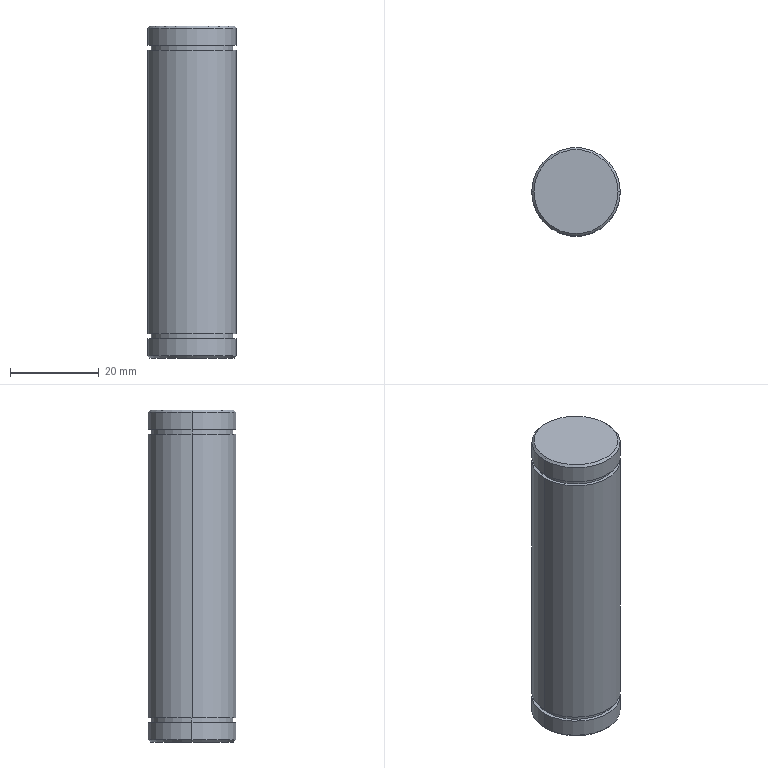Component | SolidWorks | ConnectingPin2-1 | 1 solid | 20 faces | box 20 x 20 x 75 mm | volume 23447 mm3 | cylinder 10 | plane 6 | cone 4 | commonest cylinder face diameters 20 x6 18.5 x4
build123d program:
from build123d import *

# Parameters (mm, degrees)
SKETCH1_R           = 10
BOSS_EXTRUDE1_DEPTH = 37.5
SKETCH2_W           = 1.1
SKETCH2_H           = 0.75
CHAMFER1_SIZE       = 0.5


with BuildPart() as part:
    # Sketch1 → Boss-Extrude1 (new, symmetric)
    with BuildSketch(Plane(origin=(0, 0, 0), x_dir=(0, 0, -1), z_dir=(1, 0, 0))):
        Circle(SKETCH1_R)
    extrude(amount=BOSS_EXTRUDE1_DEPTH, both=True)

    # Sketch2 → Cut-Revolve1 (revolve, cut)
    with BuildSketch(Plane.XY, mode=Mode.PRIVATE) as cut_revolve1_sk:
        with Locations((-32.55, 9.625)):
            Rectangle(SKETCH2_W, SKETCH2_H)
    cut_revolve1 = revolve(cut_revolve1_sk.sketch.rotate(Axis((37.5, 0, 0), (-1, 0, 0)), 90), axis=Axis((37.5, 0, 0), (-1, 0, 0)), mode=Mode.SUBTRACT)

    # Chamfer1
    chamfer1_edges = [part.edges().sort_by_distance(p)[0] for p in [
        (-37.5, 0, 10),
        (37.5, 0, 10),
    ]]
    chamfer(chamfer1_edges, length=CHAMFER1_SIZE)

    # Mirror4: Cut-Revolve1 across plane
    add(cut_revolve1.mirror(Plane(origin=(0, 0, 0), x_dir=(0, 0, 1), z_dir=(1, 0, 0))), mode=Mode.SUBTRACT)


solid = part.part

# Placed as in the assembly
solid = solid.moved(Location((-132.772, 396.234, 900), (0, 90, 0)))
STEP:
#1=COLOUR_RGB('',0.7922,0.8196,0.9333);
#2=FILL_AREA_STYLE_COLOUR('',#1);
#3=FILL_AREA_STYLE('',(#2));
#4=SURFACE_STYLE_FILL_AREA(#3);
#5=SURFACE_SIDE_STYLE('',(#4));
#6=SURFACE_STYLE_USAGE(.BOTH.,#5);
#7=PRESENTATION_STYLE_ASSIGNMENT((#6));
#8=CARTESIAN_POINT('',(-5.621,15.6,36.89));
#9=VERTEX_POINT('',#8);
#10=CARTESIAN_POINT('',(-4.834,15.6,36.89));
#11=VERTEX_POINT('',#10);
#12=CARTESIAN_POINT('',(-5.227,15.6,36.89));
#13=DIRECTION('',(-0.,0.,-1.));
#14=DIRECTION('',(1.,-0.,0.));
#15=AXIS2_PLACEMENT_3D('',#12,#13,#14);
#16=CIRCLE('',#15,0.3937);
#17=EDGE_CURVE('',#9,#11,#16,.T.);
#18=ORIENTED_EDGE('',*,*,#17,.T.);
#19=CARTESIAN_POINT('',(-4.834,15.6,36.736));
#20=VERTEX_POINT('',#19);
#21=CARTESIAN_POINT('',(-4.834,15.6,36.909));
#22=DIRECTION('',(-0.,0.,-1.));
#23=VECTOR('',#22,39.37);
#24=LINE('',#21,#23);
#25=EDGE_CURVE('',#11,#20,#24,.T.);
#26=ORIENTED_EDGE('',*,*,#25,.T.);
#27=CARTESIAN_POINT('',(-5.621,15.6,36.736));
#28=VERTEX_POINT('',#27);
#29=CARTESIAN_POINT('',(-5.227,15.6,36.736));
#30=DIRECTION('',(0.,-0.,1.));
#31=DIRECTION('',(1.,0.,0.));
#32=AXIS2_PLACEMENT_3D('',#29,#30,#31);
#33=CIRCLE('',#32,0.3937);
#34=EDGE_CURVE('',#20,#28,#33,.T.);
#35=ORIENTED_EDGE('',*,*,#34,.T.);
#36=CARTESIAN_POINT('',(-5.621,15.6,36.909));
#37=DIRECTION('',(-0.,0.,-1.));
#38=VECTOR('',#37,39.37);
#39=LINE('',#36,#38);
#40=EDGE_CURVE('',#9,#28,#39,.T.);
#41=ORIENTED_EDGE('',*,*,#40,.F.);
#42=EDGE_LOOP('',(#18,#26,#35,#41));
#43=FACE_OUTER_BOUND('',#42,.T.);
#44=CARTESIAN_POINT('',(-5.227,15.6,36.909));
#45=DIRECTION('',(-0.,0.,-1.));
#46=DIRECTION('',(-1.,0.,0.));
#47=AXIS2_PLACEMENT_3D('',#44,#45,#46);
#48=CYLINDRICAL_SURFACE('',#47,0.3937);
#49=ADVANCED_FACE('',(#43),#48,.T.);
#50=CARTESIAN_POINT('',(-4.853,15.6,36.909));
#51=VERTEX_POINT('',#50);
#52=CARTESIAN_POINT('',(-5.601,15.6,36.909));
#53=VERTEX_POINT('',#52);
#54=CARTESIAN_POINT('',(-5.227,15.6,36.909));
#55=DIRECTION('',(0.,-0.,1.));
#56=DIRECTION('',(1.,0.,0.));
#57=AXIS2_PLACEMENT_3D('',#54,#55,#56);
#58=CIRCLE('',#57,0.374);
#59=EDGE_CURVE('',#51,#53,#58,.T.);
#60=ORIENTED_EDGE('',*,*,#59,.F.);
#61=CARTESIAN_POINT('',(-4.853,15.6,36.909));
#62=DIRECTION('',(0.7071,0.,-0.7071));
#63=VECTOR('',#62,39.37);
#64=LINE('',#61,#63);
#65=EDGE_CURVE('',#51,#11,#64,.T.);
#66=ORIENTED_EDGE('',*,*,#65,.T.);
#67=ORIENTED_EDGE('',*,*,#17,.F.);
#68=CARTESIAN_POINT('',(-5.601,15.6,36.909));
#69=DIRECTION('',(-0.7071,0.,-0.7071));
#70=VECTOR('',#69,39.37);
#71=LINE('',#68,#70);
#72=EDGE_CURVE('',#53,#9,#71,.T.);
#73=ORIENTED_EDGE('',*,*,#72,.F.);
#74=EDGE_LOOP('',(#60,#66,#67,#73));
#75=FACE_OUTER_BOUND('',#74,.T.);
#76=CARTESIAN_POINT('',(-5.227,15.6,36.909));
#77=DIRECTION('',(-0.,0.,-1.));
#78=DIRECTION('',(-1.,0.,0.));
#79=AXIS2_PLACEMENT_3D('',#76,#77,#78);
#80=CONICAL_SURFACE('',#79,0.374,0.7854);
#81=ADVANCED_FACE('',(#75),#80,.T.);
#82=CARTESIAN_POINT('',(-5.591,15.6,36.736));
#83=VERTEX_POINT('',#82);
#84=CARTESIAN_POINT('',(-4.863,15.6,36.736));
#85=VERTEX_POINT('',#84);
#86=CARTESIAN_POINT('',(-5.227,15.6,36.736));
#87=DIRECTION('',(0.,-0.,1.));
#88=DIRECTION('',(1.,0.,0.));
#89=AXIS2_PLACEMENT_3D('',#86,#87,#88);
#90=CIRCLE('',#89,0.3642);
#91=EDGE_CURVE('',#83,#85,#90,.T.);
#92=ORIENTED_EDGE('',*,*,#91,.F.);
#93=CARTESIAN_POINT('',(-5.591,15.6,36.693));
#94=VERTEX_POINT('',#93);
#95=CARTESIAN_POINT('',(-5.591,15.6,36.736));
#96=DIRECTION('',(-0.,0.,-1.));
#97=VECTOR('',#96,39.37);
#98=LINE('',#95,#97);
#99=EDGE_CURVE('',#83,#94,#98,.T.);
#100=ORIENTED_EDGE('',*,*,#99,.T.);
#101=CARTESIAN_POINT('',(-4.863,15.6,36.693));
#102=VERTEX_POINT('',#101);
#103=CARTESIAN_POINT('',(-5.227,15.6,36.693));
#104=DIRECTION('',(0.,-0.,1.));
#105=DIRECTION('',(1.,0.,0.));
#106=AXIS2_PLACEMENT_3D('',#103,#104,#105);
#107=CIRCLE('',#106,0.3642);
#108=EDGE_CURVE('',#94,#102,#107,.T.);
#109=ORIENTED_EDGE('',*,*,#108,.T.);
#110=CARTESIAN_POINT('',(-4.863,15.6,36.736));
#111=DIRECTION('',(-0.,0.,-1.));
#112=VECTOR('',#111,39.37);
#113=LINE('',#110,#112);
#114=EDGE_CURVE('',#85,#102,#113,.T.);
#115=ORIENTED_EDGE('',*,*,#114,.F.);
#116=EDGE_LOOP('',(#92,#100,#109,#115));
#117=FACE_OUTER_BOUND('',#116,.T.);
#118=CARTESIAN_POINT('',(-5.227,15.6,36.736));
#119=DIRECTION('',(-0.,0.,-1.));
#120=DIRECTION('',(1.,0.,0.));
#121=AXIS2_PLACEMENT_3D('',#118,#119,#120);
#122=CYLINDRICAL_SURFACE('',#121,0.3642);
#123=ADVANCED_FACE('',(#117),#122,.T.);
#124=CARTESIAN_POINT('',(-5.601,15.6,33.957));
#125=VERTEX_POINT('',#124);
#126=CARTESIAN_POINT('',(-4.853,15.6,33.957));
#127=VERTEX_POINT('',#126);
#128=CARTESIAN_POINT('',(-5.227,15.6,33.957));
#129=DIRECTION('',(-0.,0.,-1.));
#130=DIRECTION('',(1.,-0.,0.));
#131=AXIS2_PLACEMENT_3D('',#128,#129,#130);
#132=CIRCLE('',#131,0.374);
#133=EDGE_CURVE('',#125,#127,#132,.T.);
#134=ORIENTED_EDGE('',*,*,#133,.F.);
#135=CARTESIAN_POINT('',(-5.621,15.6,33.976));
#136=VERTEX_POINT('',#135);
#137=CARTESIAN_POINT('',(-5.621,15.6,33.976));
#138=DIRECTION('',(-0.7071,0.,0.7071));
#139=VECTOR('',#138,39.37);
#140=LINE('',#137,#139);
#141=EDGE_CURVE('',#125,#136,#140,.T.);
#142=ORIENTED_EDGE('',*,*,#141,.T.);
#143=CARTESIAN_POINT('',(-4.834,15.6,33.976));
#144=VERTEX_POINT('',#143);
#145=CARTESIAN_POINT('',(-5.227,15.6,33.976));
#146=DIRECTION('',(0.,-0.,1.));
#147=DIRECTION('',(1.,0.,0.));
#148=AXIS2_PLACEMENT_3D('',#145,#146,#147);
#149=CIRCLE('',#148,0.3937);
#150=EDGE_CURVE('',#144,#136,#149,.T.);
#151=ORIENTED_EDGE('',*,*,#150,.F.);
#152=CARTESIAN_POINT('',(-4.834,15.6,33.976));
#153=DIRECTION('',(0.7071,-0.,0.7071));
#154=VECTOR('',#153,39.37);
#155=LINE('',#152,#154);
#156=EDGE_CURVE('',#127,#144,#155,.T.);
#157=ORIENTED_EDGE('',*,*,#156,.F.);
#158=EDGE_LOOP('',(#134,#142,#151,#157));
#159=FACE_OUTER_BOUND('',#158,.T.);
#160=CARTESIAN_POINT('',(-5.227,15.6,33.976));
#161=DIRECTION('',(0.,-0.,1.));
#162=DIRECTION('',(1.,0.,0.));
#163=AXIS2_PLACEMENT_3D('',#160,#161,#162);
#164=CONICAL_SURFACE('',#163,0.3937,0.7854);
#165=ADVANCED_FACE('',(#159),#164,.T.);
#166=CARTESIAN_POINT('',(-4.834,15.6,36.693));
#167=VERTEX_POINT('',#166);
#168=CARTESIAN_POINT('',(-5.621,15.6,36.693));
#169=VERTEX_POINT('',#168);
#170=CARTESIAN_POINT('',(-5.227,15.6,36.693));
#171=DIRECTION('',(0.,-0.,1.));
#172=DIRECTION('',(1.,0.,0.));
#173=AXIS2_PLACEMENT_3D('',#170,#171,#172);
#174=CIRCLE('',#173,0.3937);
#175=EDGE_CURVE('',#167,#169,#174,.T.);
#176=ORIENTED_EDGE('',*,*,#175,.F.);
#177=CARTESIAN_POINT('',(-4.834,15.6,34.173));
#178=VERTEX_POINT('',#177);
#179=CARTESIAN_POINT('',(-4.834,15.6,36.909));
#180=DIRECTION('',(-0.,0.,-1.));
#181=VECTOR('',#180,39.37);
#182=LINE('',#179,#181);
#183=EDGE_CURVE('',#167,#178,#182,.T.);
#184=ORIENTED_EDGE('',*,*,#183,.T.);
#185=CARTESIAN_POINT('',(-5.621,15.6,34.173));
#186=VERTEX_POINT('',#185);
#187=CARTESIAN_POINT('',(-5.227,15.6,34.173));
#188=DIRECTION('',(0.,-0.,1.));
#189=DIRECTION('',(1.,0.,0.));
#190=AXIS2_PLACEMENT_3D('',#187,#188,#189);
#191=CIRCLE('',#190,0.3937);
#192=EDGE_CURVE('',#178,#186,#191,.T.);
#193=ORIENTED_EDGE('',*,*,#192,.T.);
#194=CARTESIAN_POINT('',(-5.621,15.6,36.909));
#195=DIRECTION('',(-0.,0.,-1.));
#196=VECTOR('',#195,39.37);
#197=LINE('',#194,#196);
#198=EDGE_CURVE('',#169,#186,#197,.T.);
#199=ORIENTED_EDGE('',*,*,#198,.F.);
#200=EDGE_LOOP('',(#176,#184,#193,#199));
#201=FACE_OUTER_BOUND('',#200,.T.);
#202=CARTESIAN_POINT('',(-5.227,15.6,36.909));
#203=DIRECTION('',(-0.,0.,-1.));
#204=DIRECTION('',(-1.,0.,0.));
#205=AXIS2_PLACEMENT_3D('',#202,#203,#204);
#206=CYLINDRICAL_SURFACE('',#205,0.3937);
#207=ADVANCED_FACE('',(#201),#206,.T.);
#208=CARTESIAN_POINT('',(-4.863,15.6,34.13));
#209=VERTEX_POINT('',#208);
#210=CARTESIAN_POINT('',(-5.591,15.6,34.13));
#211=VERTEX_POINT('',#210);
#212=CARTESIAN_POINT('',(-5.227,15.6,34.13));
#213=DIRECTION('',(0.,-0.,1.));
#214=DIRECTION('',(1.,0.,0.));
#215=AXIS2_PLACEMENT_3D('',#212,#213,#214);
#216=CIRCLE('',#215,0.3642);
#217=EDGE_CURVE('',#209,#211,#216,.T.);
#218=ORIENTED_EDGE('',*,*,#217,.T.);
#219=CARTESIAN_POINT('',(-5.591,15.6,34.173));
#220=VERTEX_POINT('',#219);
#221=CARTESIAN_POINT('',(-5.591,15.6,36.909));
#222=DIRECTION('',(0.,-0.,1.));
#223=VECTOR('',#222,39.37);
#224=LINE('',#221,#223);
#225=EDGE_CURVE('',#211,#220,#224,.T.);
#226=ORIENTED_EDGE('',*,*,#225,.T.);
#227=CARTESIAN_POINT('',(-4.863,15.6,34.173));
#228=VERTEX_POINT('',#227);
#229=CARTESIAN_POINT('',(-5.227,15.6,34.173));
#230=DIRECTION('',(0.,-0.,1.));
#231=DIRECTION('',(1.,0.,0.));
#232=AXIS2_PLACEMENT_3D('',#229,#230,#231);
#233=CIRCLE('',#232,0.3642);
#234=EDGE_CURVE('',#228,#220,#233,.T.);
#235=ORIENTED_EDGE('',*,*,#234,.F.);
#236=CARTESIAN_POINT('',(-4.863,15.6,36.909));
#237=DIRECTION('',(0.,-0.,1.));
#238=VECTOR('',#237,39.37);
#239=LINE('',#236,#238);
#240=EDGE_CURVE('',#209,#228,#239,.T.);
#241=ORIENTED_EDGE('',*,*,#240,.F.);
#242=EDGE_LOOP('',(#218,#226,#235,#241));
#243=FACE_OUTER_BOUND('',#242,.T.);
#244=CARTESIAN_POINT('',(-5.227,15.6,36.909));
#245=DIRECTION('',(0.,-0.,1.));
#246=DIRECTION('',(1.,0.,0.));
#247=AXIS2_PLACEMENT_3D('',#244,#245,#246);
#248=CYLINDRICAL_SURFACE('',#247,0.3642);
#249=ADVANCED_FACE('',(#243),#248,.T.);
#250=CARTESIAN_POINT('',(-4.834,15.6,34.13));
#251=VERTEX_POINT('',#250);
#252=CARTESIAN_POINT('',(-5.621,15.6,34.13));
#253=VERTEX_POINT('',#252);
#254=CARTESIAN_POINT('',(-5.227,15.6,34.13));
#255=DIRECTION('',(0.,-0.,1.));
#256=DIRECTION('',(1.,0.,0.));
#257=AXIS2_PLACEMENT_3D('',#254,#255,#256);
#258=CIRCLE('',#257,0.3937);
#259=EDGE_CURVE('',#251,#253,#258,.T.);
#260=ORIENTED_EDGE('',*,*,#259,.F.);
#261=CARTESIAN_POINT('',(-4.834,15.6,36.909));
#262=DIRECTION('',(-0.,0.,-1.));
#263=VECTOR('',#262,39.37);
#264=LINE('',#261,#263);
#265=EDGE_CURVE('',#251,#144,#264,.T.);
#266=ORIENTED_EDGE('',*,*,#265,.T.);
#267=ORIENTED_EDGE('',*,*,#150,.T.);
#268=CARTESIAN_POINT('',(-5.621,15.6,36.909));
#269=DIRECTION('',(-0.,0.,-1.));
#270=VECTOR('',#269,39.37);
#271=LINE('',#268,#270);
#272=EDGE_CURVE('',#253,#136,#271,.T.);
#273=ORIENTED_EDGE('',*,*,#272,.F.);
#274=EDGE_LOOP('',(#260,#266,#267,#273));
#275=FACE_OUTER_BOUND('',#274,.T.);
#276=CARTESIAN_POINT('',(-5.227,15.6,36.909));
#277=DIRECTION('',(-0.,0.,-1.));
#278=DIRECTION('',(-1.,0.,0.));
#279=AXIS2_PLACEMENT_3D('',#276,#277,#278);
#280=CYLINDRICAL_SURFACE('',#279,0.3937);
#281=ADVANCED_FACE('',(#275),#280,.T.);
#282=ORIENTED_EDGE('',*,*,#265,.F.);
#283=CARTESIAN_POINT('',(-5.227,15.6,34.13));
#284=DIRECTION('',(0.,-0.,1.));
#285=DIRECTION('',(1.,0.,0.));
#286=AXIS2_PLACEMENT_3D('',#283,#284,#285);
#287=CIRCLE('',#286,0.3937);
#288=EDGE_CURVE('',#253,#251,#287,.T.);
#289=ORIENTED_EDGE('',*,*,#288,.F.);
#290=ORIENTED_EDGE('',*,*,#272,.T.);
#291=CARTESIAN_POINT('',(-5.227,15.6,33.976));
#292=DIRECTION('',(0.,-0.,1.));
#293=DIRECTION('',(1.,0.,0.));
#294=AXIS2_PLACEMENT_3D('',#291,#292,#293);
#295=CIRCLE('',#294,0.3937);
#296=EDGE_CURVE('',#136,#144,#295,.T.);
#297=ORIENTED_EDGE('',*,*,#296,.T.);
#298=EDGE_LOOP('',(#282,#289,#290,#297));
#299=FACE_OUTER_BOUND('',#298,.T.);
#300=CARTESIAN_POINT('',(-5.227,15.6,36.909));
#301=DIRECTION('',(-0.,0.,-1.));
#302=DIRECTION('',(-1.,0.,0.));
#303=AXIS2_PLACEMENT_3D('',#300,#301,#302);
#304=CYLINDRICAL_SURFACE('',#303,0.3937);
#305=ADVANCED_FACE('',(#299),#304,.T.);
#306=CARTESIAN_POINT('',(-5.227,15.6,33.957));
#307=DIRECTION('',(-0.,0.,-1.));
#308=DIRECTION('',(1.,-0.,0.));
#309=AXIS2_PLACEMENT_3D('',#306,#307,#308);
#310=CIRCLE('',#309,0.374);
#311=EDGE_CURVE('',#127,#125,#310,.T.);
#312=ORIENTED_EDGE('',*,*,#311,.T.);
#313=ORIENTED_EDGE('',*,*,#133,.T.);
#314=EDGE_LOOP('',(#312,#313));
#315=FACE_OUTER_BOUND('',#314,.T.);
#316=CARTESIAN_POINT('',(-5.227,15.6,33.957));
#317=DIRECTION('',(0.,-0.,1.));
#318=DIRECTION('',(1.,-0.,-0.));
#319=AXIS2_PLACEMENT_3D('',#316,#317,#318);
#320=PLANE('',#319);
#321=ADVANCED_FACE('',(#315),#320,.F.);
#322=ORIENTED_EDGE('',*,*,#217,.F.);
#323=CARTESIAN_POINT('',(-5.227,15.6,34.13));
#324=DIRECTION('',(0.,-0.,1.));
#325=DIRECTION('',(1.,0.,0.));
#326=AXIS2_PLACEMENT_3D('',#323,#324,#325);
#327=CIRCLE('',#326,0.3642);
#328=EDGE_CURVE('',#211,#209,#327,.T.);
#329=ORIENTED_EDGE('',*,*,#328,.F.);
#330=EDGE_LOOP('',(#322,#329));
#331=FACE_BOUND('',#330,.T.);
#332=ORIENTED_EDGE('',*,*,#288,.T.);
#333=ORIENTED_EDGE('',*,*,#259,.T.);
#334=EDGE_LOOP('',(#332,#333));
#335=FACE_OUTER_BOUND('',#334,.T.);
#336=CARTESIAN_POINT('',(-5.227,15.993,34.13));
#337=DIRECTION('',(-0.,0.,-1.));
#338=DIRECTION('',(-1.,0.,0.));
#339=AXIS2_PLACEMENT_3D('',#336,#337,#338);
#340=PLANE('',#339);
#341=ADVANCED_FACE('',(#331,#335),#340,.F.);
#342=ORIENTED_EDGE('',*,*,#225,.F.);
#343=ORIENTED_EDGE('',*,*,#328,.T.);
#344=ORIENTED_EDGE('',*,*,#240,.T.);
#345=CARTESIAN_POINT('',(-5.227,15.6,34.173));
#346=DIRECTION('',(0.,-0.,1.));
#347=DIRECTION('',(1.,0.,0.));
#348=AXIS2_PLACEMENT_3D('',#345,#346,#347);
#349=CIRCLE('',#348,0.3642);
#350=EDGE_CURVE('',#220,#228,#349,.T.);
#351=ORIENTED_EDGE('',*,*,#350,.F.);
#352=EDGE_LOOP('',(#342,#343,#344,#351));
#353=FACE_OUTER_BOUND('',#352,.T.);
#354=CARTESIAN_POINT('',(-5.227,15.6,36.909));
#355=DIRECTION('',(0.,-0.,1.));
#356=DIRECTION('',(1.,0.,0.));
#357=AXIS2_PLACEMENT_3D('',#354,#355,#356);
#358=CYLINDRICAL_SURFACE('',#357,0.3642);
#359=ADVANCED_FACE('',(#353),#358,.T.);
#360=CARTESIAN_POINT('',(-5.227,15.6,34.173));
#361=DIRECTION('',(0.,-0.,1.));
#362=DIRECTION('',(1.,0.,0.));
#363=AXIS2_PLACEMENT_3D('',#360,#361,#362);
#364=CIRCLE('',#363,0.3937);
#365=EDGE_CURVE('',#186,#178,#364,.T.);
#366=ORIENTED_EDGE('',*,*,#365,.F.);
#367=ORIENTED_EDGE('',*,*,#192,.F.);
#368=EDGE_LOOP('',(#366,#367));
#369=FACE_OUTER_BOUND('',#368,.T.);
#370=ORIENTED_EDGE('',*,*,#234,.T.);
#371=ORIENTED_EDGE('',*,*,#350,.T.);
#372=EDGE_LOOP('',(#370,#371));
#373=FACE_BOUND('',#372,.T.);
#374=CARTESIAN_POINT('',(-5.227,15.993,34.173));
#375=DIRECTION('',(0.,-0.,1.));
#376=DIRECTION('',(1.,-0.,-0.));
#377=AXIS2_PLACEMENT_3D('',#374,#375,#376);
#378=PLANE('',#377);
#379=ADVANCED_FACE('',(#369,#373),#378,.F.);
#380=ORIENTED_EDGE('',*,*,#183,.F.);
#381=CARTESIAN_POINT('',(-5.227,15.6,36.693));
#382=DIRECTION('',(0.,-0.,1.));
#383=DIRECTION('',(1.,0.,0.));
#384=AXIS2_PLACEMENT_3D('',#381,#382,#383);
#385=CIRCLE('',#384,0.3937);
#386=EDGE_CURVE('',#169,#167,#385,.T.);
#387=ORIENTED_EDGE('',*,*,#386,.F.);
#388=ORIENTED_EDGE('',*,*,#198,.T.);
#389=ORIENTED_EDGE('',*,*,#365,.T.);
#390=EDGE_LOOP('',(#380,#387,#388,#389));
#391=FACE_OUTER_BOUND('',#390,.T.);
#392=CARTESIAN_POINT('',(-5.227,15.6,36.909));
#393=DIRECTION('',(-0.,0.,-1.));
#394=DIRECTION('',(-1.,0.,0.));
#395=AXIS2_PLACEMENT_3D('',#392,#393,#394);
#396=CYLINDRICAL_SURFACE('',#395,0.3937);
#397=ADVANCED_FACE('',(#391),#396,.T.);
#398=ORIENTED_EDGE('',*,*,#141,.F.);
#399=ORIENTED_EDGE('',*,*,#311,.F.);
#400=ORIENTED_EDGE('',*,*,#156,.T.);
#401=ORIENTED_EDGE('',*,*,#296,.F.);
#402=EDGE_LOOP('',(#398,#399,#400,#401));
#403=FACE_OUTER_BOUND('',#402,.T.);
#404=CARTESIAN_POINT('',(-5.227,15.6,33.976));
#405=DIRECTION('',(0.,-0.,1.));
#406=DIRECTION('',(1.,0.,0.));
#407=AXIS2_PLACEMENT_3D('',#404,#405,#406);
#408=CONICAL_SURFACE('',#407,0.3937,0.7854);
#409=ADVANCED_FACE('',(#403),#408,.T.);
#410=CARTESIAN_POINT('',(-5.227,15.6,36.736));
#411=DIRECTION('',(0.,-0.,1.));
#412=DIRECTION('',(1.,0.,0.));
#413=AXIS2_PLACEMENT_3D('',#410,#411,#412);
#414=CIRCLE('',#413,0.3642);
#415=EDGE_CURVE('',#85,#83,#414,.T.);
#416=ORIENTED_EDGE('',*,*,#415,.T.);
#417=ORIENTED_EDGE('',*,*,#91,.T.);
#418=EDGE_LOOP('',(#416,#417));
#419=FACE_BOUND('',#418,.T.);
#420=CARTESIAN_POINT('',(-5.227,15.6,36.736));
#421=DIRECTION('',(0.,-0.,1.));
#422=DIRECTION('',(1.,0.,0.));
#423=AXIS2_PLACEMENT_3D('',#420,#421,#422);
#424=CIRCLE('',#423,0.3937);
#425=EDGE_CURVE('',#28,#20,#424,.T.);
#426=ORIENTED_EDGE('',*,*,#425,.F.);
#427=ORIENTED_EDGE('',*,*,#34,.F.);
#428=EDGE_LOOP('',(#426,#427));
#429=FACE_OUTER_BOUND('',#428,.T.);
#430=CARTESIAN_POINT('',(-5.227,15.993,36.736));
#431=DIRECTION('',(0.,-0.,1.));
#432=DIRECTION('',(-1.,0.,0.));
#433=AXIS2_PLACEMENT_3D('',#430,#431,#432);
#434=PLANE('',#433);
#435=ADVANCED_FACE('',(#419,#429),#434,.F.);
#436=ORIENTED_EDGE('',*,*,#99,.F.);
#437=ORIENTED_EDGE('',*,*,#415,.F.);
#438=ORIENTED_EDGE('',*,*,#114,.T.);
#439=CARTESIAN_POINT('',(-5.227,15.6,36.693));
#440=DIRECTION('',(0.,-0.,1.));
#441=DIRECTION('',(1.,0.,0.));
#442=AXIS2_PLACEMENT_3D('',#439,#440,#441);
#443=CIRCLE('',#442,0.3642);
#444=EDGE_CURVE('',#102,#94,#443,.T.);
#445=ORIENTED_EDGE('',*,*,#444,.T.);
#446=EDGE_LOOP('',(#436,#437,#438,#445));
#447=FACE_OUTER_BOUND('',#446,.T.);
#448=CARTESIAN_POINT('',(-5.227,15.6,36.736));
#449=DIRECTION('',(-0.,0.,-1.));
#450=DIRECTION('',(1.,0.,0.));
#451=AXIS2_PLACEMENT_3D('',#448,#449,#450);
#452=CYLINDRICAL_SURFACE('',#451,0.3642);
#453=ADVANCED_FACE('',(#447),#452,.T.);
#454=ORIENTED_EDGE('',*,*,#386,.T.);
#455=ORIENTED_EDGE('',*,*,#175,.T.);
#456=EDGE_LOOP('',(#454,#455));
#457=FACE_OUTER_BOUND('',#456,.T.);
#458=ORIENTED_EDGE('',*,*,#444,.F.);
#459=ORIENTED_EDGE('',*,*,#108,.F.);
#460=EDGE_LOOP('',(#458,#459));
#461=FACE_BOUND('',#460,.T.);
#462=CARTESIAN_POINT('',(-5.227,15.993,36.693));
#463=DIRECTION('',(-0.,0.,-1.));
#464=DIRECTION('',(1.,-0.,-0.));
#465=AXIS2_PLACEMENT_3D('',#462,#463,#464);
#466=PLANE('',#465);
#467=ADVANCED_FACE('',(#457,#461),#466,.F.);
#468=CARTESIAN_POINT('',(-5.227,15.6,36.909));
#469=DIRECTION('',(0.,-0.,1.));
#470=DIRECTION('',(1.,0.,0.));
#471=AXIS2_PLACEMENT_3D('',#468,#469,#470);
#472=CIRCLE('',#471,0.374);
#473=EDGE_CURVE('',#53,#51,#472,.T.);
#474=ORIENTED_EDGE('',*,*,#473,.T.);
#475=ORIENTED_EDGE('',*,*,#59,.T.);
#476=EDGE_LOOP('',(#474,#475));
#477=FACE_OUTER_BOUND('',#476,.T.);
#478=CARTESIAN_POINT('',(-5.227,15.6,36.909));
#479=DIRECTION('',(0.,-0.,1.));
#480=DIRECTION('',(1.,-0.,-0.));
#481=AXIS2_PLACEMENT_3D('',#478,#479,#480);
#482=PLANE('',#481);
#483=ADVANCED_FACE('',(#477),#482,.T.);
#484=ORIENTED_EDGE('',*,*,#65,.F.);
#485=ORIENTED_EDGE('',*,*,#473,.F.);
#486=ORIENTED_EDGE('',*,*,#72,.T.);
#487=CARTESIAN_POINT('',(-5.227,15.6,36.89));
#488=DIRECTION('',(-0.,0.,-1.));
#489=DIRECTION('',(1.,-0.,0.));
#490=AXIS2_PLACEMENT_3D('',#487,#488,#489);
#491=CIRCLE('',#490,0.3937);
#492=EDGE_CURVE('',#11,#9,#491,.T.);
#493=ORIENTED_EDGE('',*,*,#492,.F.);
#494=EDGE_LOOP('',(#484,#485,#486,#493));
#495=FACE_OUTER_BOUND('',#494,.T.);
#496=CARTESIAN_POINT('',(-5.227,15.6,36.909));
#497=DIRECTION('',(-0.,0.,-1.));
#498=DIRECTION('',(-1.,0.,0.));
#499=AXIS2_PLACEMENT_3D('',#496,#497,#498);
#500=CONICAL_SURFACE('',#499,0.374,0.7854);
#501=ADVANCED_FACE('',(#495),#500,.T.);
#502=ORIENTED_EDGE('',*,*,#25,.F.);
#503=ORIENTED_EDGE('',*,*,#492,.T.);
#504=ORIENTED_EDGE('',*,*,#40,.T.);
#505=ORIENTED_EDGE('',*,*,#425,.T.);
#506=EDGE_LOOP('',(#502,#503,#504,#505));
#507=FACE_OUTER_BOUND('',#506,.T.);
#508=CARTESIAN_POINT('',(-5.227,15.6,36.909));
#509=DIRECTION('',(-0.,0.,-1.));
#510=DIRECTION('',(-1.,0.,0.));
#511=AXIS2_PLACEMENT_3D('',#508,#509,#510);
#512=CYLINDRICAL_SURFACE('',#511,0.3937);
#513=ADVANCED_FACE('',(#507),#512,.T.);
#514=CLOSED_SHELL('',(#49,#81,#123,#165,#207,#249,#281,#305,#321,#341,#359,#379,#397,#409,#435,#453,#467,#483,#501,#513));
#515=MANIFOLD_SOLID_BREP('',#514);
#516=STYLED_ITEM('',(#7),#515);
#517=PRESENTATION_LAYER_ASSIGNMENT('','',(#516));
#518=(LENGTH_UNIT()NAMED_UNIT(*)SI_UNIT($,.METRE.));
#519=LENGTH_MEASURE_WITH_UNIT(LENGTH_MEASURE(0.0254),#518);
#520=DIMENSIONAL_EXPONENTS(1.,0.,0.,0.,0.,0.,0.);
#521=(CONVERSION_BASED_UNIT('',#519)LENGTH_UNIT()NAMED_UNIT(#520));
#522=UNCERTAINTY_MEASURE_WITH_UNIT(LENGTH_MEASURE(0.00001),#521,'','');
#523=(NAMED_UNIT(*)PLANE_ANGLE_UNIT()SI_UNIT($,.RADIAN.));
#524=(NAMED_UNIT(*)SI_UNIT($,.STERADIAN.)SOLID_ANGLE_UNIT());
#525=(GEOMETRIC_REPRESENTATION_CONTEXT(3)GLOBAL_UNCERTAINTY_ASSIGNED_CONTEXT((#522))GLOBAL_UNIT_ASSIGNED_CONTEXT((#521,#523,#524))REPRESENTATION_CONTEXT('',''));
#526=MECHANICAL_DESIGN_GEOMETRIC_PRESENTATION_REPRESENTATION('',(#516),#525);
#527=CARTESIAN_POINT('',(0.,0.,0.));
#528=DIRECTION('',(0.,0.,1.));
#529=DIRECTION('',(1.,0.,0.));
#530=AXIS2_PLACEMENT_3D('',#527,#528,#529);
#531=(LENGTH_UNIT()NAMED_UNIT(*)SI_UNIT($,.METRE.));
#532=LENGTH_MEASURE_WITH_UNIT(LENGTH_MEASURE(0.0254),#531);
#533=DIMENSIONAL_EXPONENTS(1.,0.,0.,0.,0.,0.,0.);
#534=(CONVERSION_BASED_UNIT('',#532)LENGTH_UNIT()NAMED_UNIT(#533));
#535=UNCERTAINTY_MEASURE_WITH_UNIT(LENGTH_MEASURE(0.00001),#534,'','');
#536=(NAMED_UNIT(*)PLANE_ANGLE_UNIT()SI_UNIT($,.RADIAN.));
#537=(NAMED_UNIT(*)SI_UNIT($,.STERADIAN.)SOLID_ANGLE_UNIT());
#538=(GEOMETRIC_REPRESENTATION_CONTEXT(3)GLOBAL_UNCERTAINTY_ASSIGNED_CONTEXT((#535))GLOBAL_UNIT_ASSIGNED_CONTEXT((#534,#536,#537))REPRESENTATION_CONTEXT('',''));
#539=ADVANCED_BREP_SHAPE_REPRESENTATION('',(#515,#530),#538);